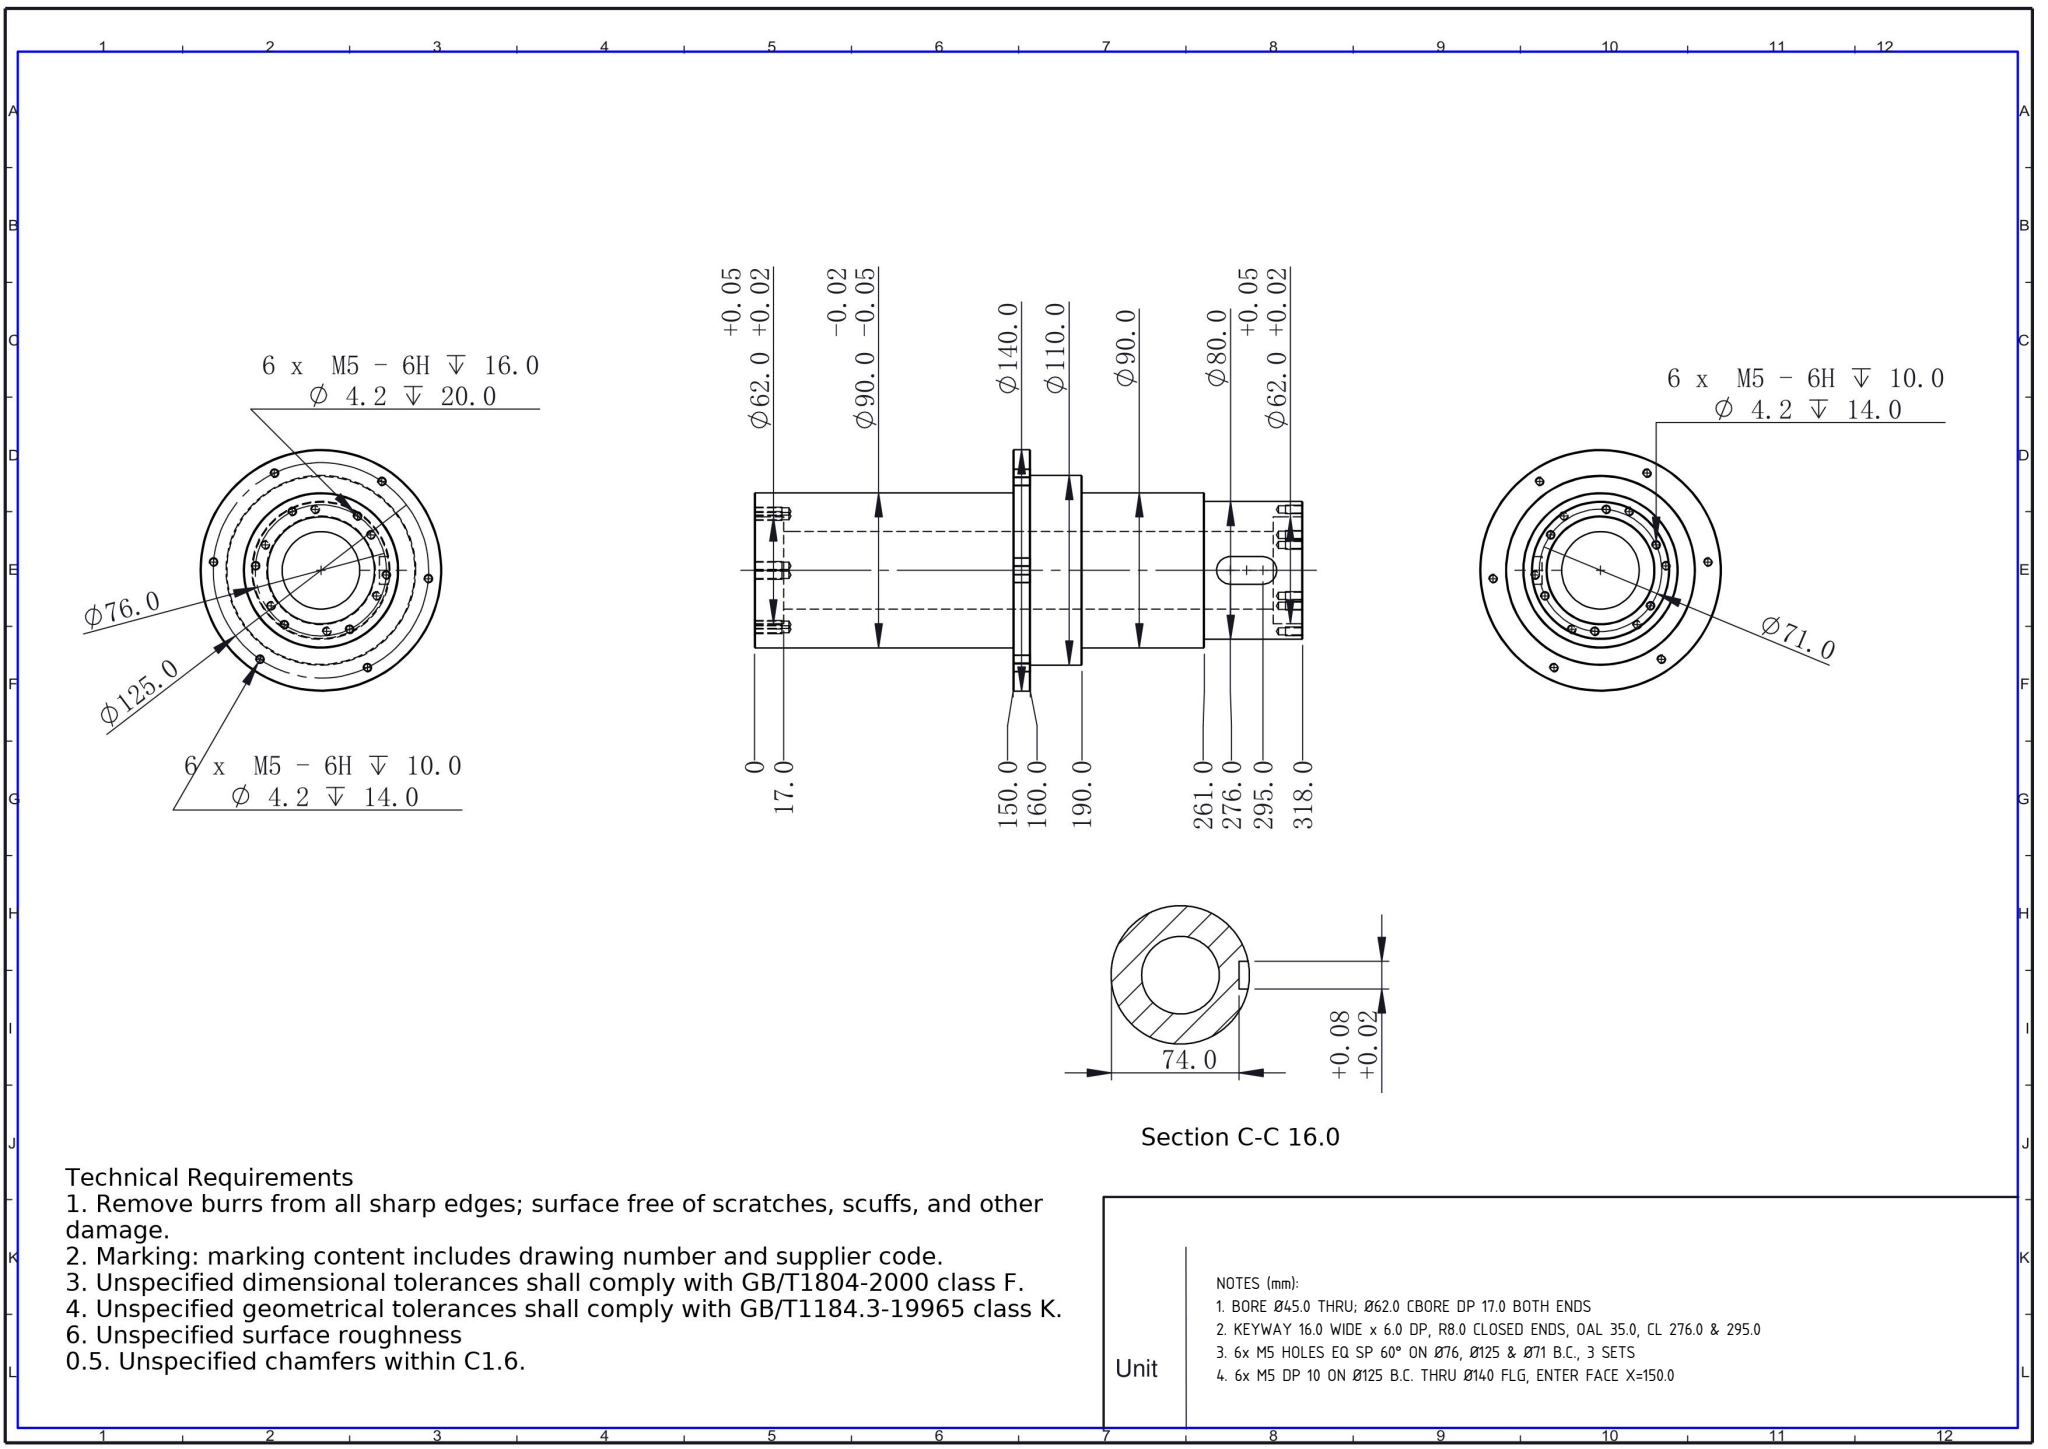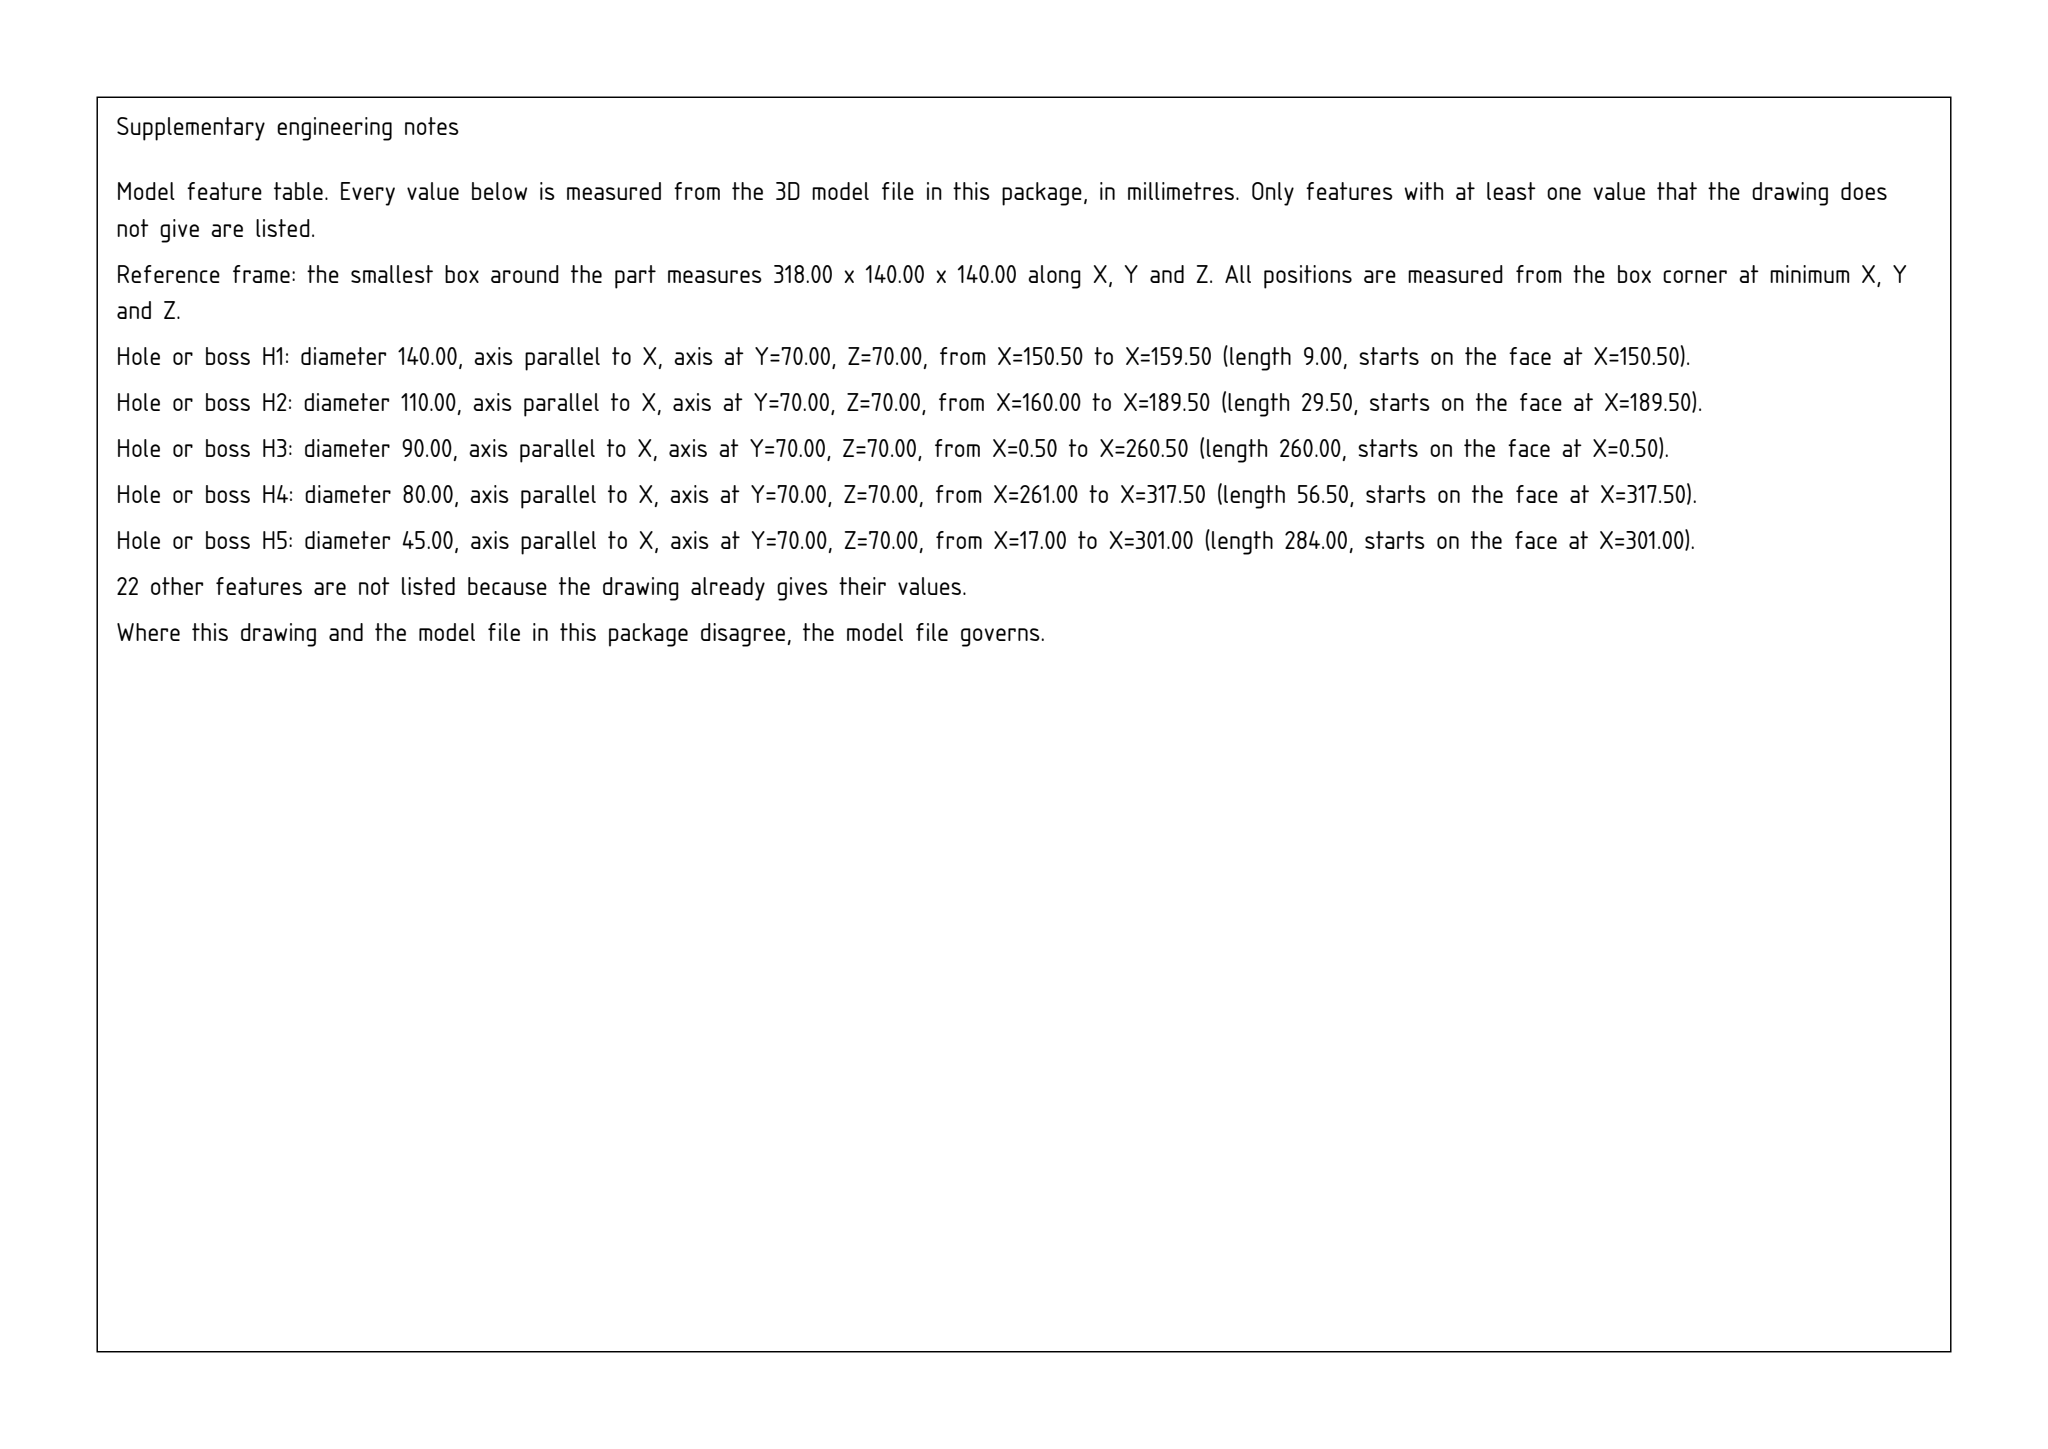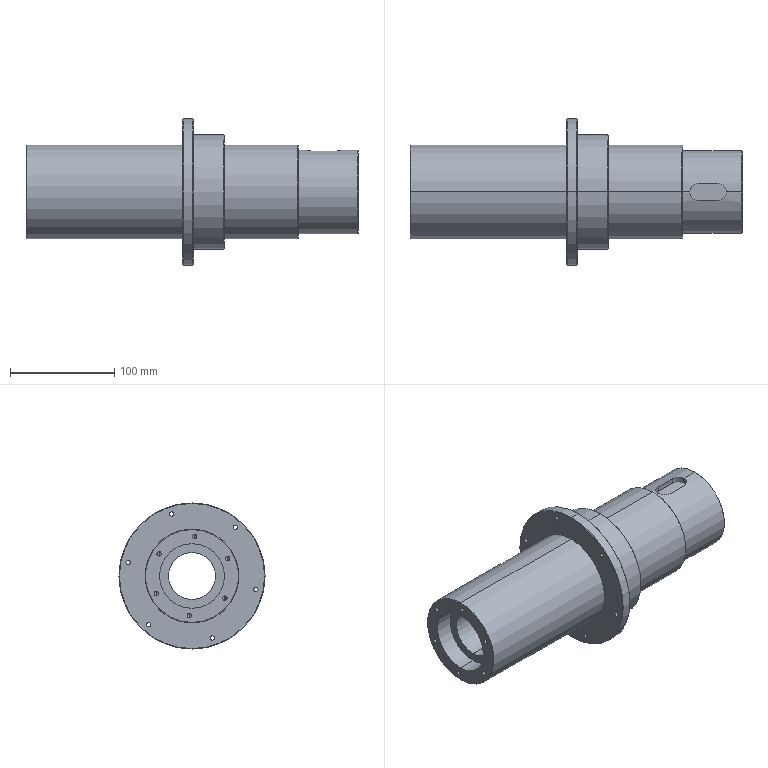Part | SolidWorks | mm | 1 solid | 104 faces | box 318 x 140 x 140 mm | volume 1570246 mm3 | cylinder 55 | cone 38 | plane 11 | commonest cylinder face diameters 4.2 x36 62 x4 90 x4 16 x3 80 x2 110 x2 140 x2 45 x2
Drawing notes:
BORE Ø45.0 THRU; Ø62.0 CBORE DP 17.0 BOTH ENDS | from the solid: Ø45 x-cyl len 284 (x=17 to 301); Ø62 x-cyls at both ends; x-planes 0,17,301,318
KEYWAY 16.0 WIDE x 6.0 DP, R8.0 CLOSED ENDS, OAL 35.0, CL 276.0 & 295.0 | from the solid: y-planes 62.0/78.0 = 16 wide; z-plane 104.0 floor vs Ø80 axis z=70 -> 6 DP; Ø16 z-cyls len 6.0 at x=276.0 & 295.0 -> 19+16=35 OAL
6x M5 HOLES EQ SP 60° ON Ø76, Ø125 & Ø71 B.C., 3 SETS | from the solid: Ø4.2 groups of 6: L=20 at r=38.0, L=10 at r=62.5, L=14 at r=35.5, all 60° increments about axis y=z=70
6x M5 DP 10 ON Ø125 B.C. THRU Ø140 FLG, ENTER FACE X=150.0 | from the solid: Ø4.2 L=10.0 holes at r=62.5 lie in Ø140 flange between x-planes 150.0 and 160.0; hole len = flange thk
build123d program:
from build123d import *

# Parameters (mm, degrees)
CUT_EXTRUDE1_DEPTH    = 6
M5_TAPPED_HOLE1_D     = 4.2
M5_TAPPED_HOLE1_DEPTH = 14
M5_TAPPED_HOLE1_TIP   = 1.262
M5_TAPPED_HOLE2_D     = 4.2
M5_TAPPED_HOLE2_DEPTH = 14
M5_TAPPED_HOLE2_TIP   = 1.262
M5_TAPPED_HOLE3_D     = 4.2
M5_TAPPED_HOLE3_DEPTH = 20
M5_TAPPED_HOLE3_TIP   = 1.262
CHAMFER1_SIZE         = 0.5


with BuildPart() as part:
    # Sketch1 → Revolve1 (revolve)
    with BuildSketch(Plane.XY, mode=Mode.PRIVATE) as revolve1_sk:
        Polygon((17, 22.5), (17, 31), (0, 31), (0, 45), (150, 45), (150, 70), (160, 70), (160, 55), (190, 55), (190, 45), (261, 45), (261, 40), (318, 40), (318, 31), (301, 31), (301, 22.5), align=None)
    revolve(revolve1_sk.sketch.rotate(Axis((0, 0, 0), (1, 0, 0)), 90), axis=Axis((0, 0, 0), (1, 0, 0)))

    # Sketch2 → Cut-Extrude1 (cut)
    with BuildSketch(Plane.XY.offset(40)):
        with BuildLine():
            Line((276, 8), (295, 8))
            ThreePointArc((295, 8), (303, 0), (295, -8))
            Line((295, -8), (276, -8))
            ThreePointArc((276, -8), (268, 0), (276, 8))
        make_face()
    extrude(amount=-CUT_EXTRUDE1_DEPTH, mode=Mode.SUBTRACT)

    # M5 Tapped Hole1
    with Locations(Plane(origin=(318, 0, 0), x_dir=(0, 0, -1), z_dir=(1, 0, 0))):
        with Locations((-32.272, -14.791), (-28.945, 20.553), (3.327, 35.344), (32.272, 14.791), (28.945, -20.553), (-3.327, -35.344)):
            Hole(M5_TAPPED_HOLE1_D / 2, depth=M5_TAPPED_HOLE1_DEPTH)
            with Locations((0, 0, -(M5_TAPPED_HOLE1_DEPTH + M5_TAPPED_HOLE1_TIP / 2))):  # 118° drill point
                Cone(0, M5_TAPPED_HOLE1_D / 2, M5_TAPPED_HOLE1_TIP, mode=Mode.SUBTRACT)

    # M5 Tapped Hole2
    with Locations(Plane.ZY.offset(-150)):
        with Locations((46.627, -41.62), (59.357, 19.57), (12.73, 61.19), (-46.627, 41.62), (-59.357, -19.57), (-12.73, -61.19)):
            Hole(M5_TAPPED_HOLE2_D / 2, depth=M5_TAPPED_HOLE2_DEPTH)
            with Locations((0, 0, -(M5_TAPPED_HOLE2_DEPTH + M5_TAPPED_HOLE2_TIP / 2))):  # 118° drill point
                Cone(0, M5_TAPPED_HOLE2_D / 2, M5_TAPPED_HOLE2_TIP, mode=Mode.SUBTRACT)

    # M5 Tapped Hole3
    with Locations(Plane.ZY):
        with Locations((-16.661, 34.153), (-37.908, 2.647), (21.246, 31.506), (37.908, -2.647), (16.661, -34.153), (-21.246, -31.506)):
            Hole(M5_TAPPED_HOLE3_D / 2, depth=M5_TAPPED_HOLE3_DEPTH)
            with Locations((0, 0, -(M5_TAPPED_HOLE3_DEPTH + M5_TAPPED_HOLE3_TIP / 2))):  # 118° drill point
                Cone(0, M5_TAPPED_HOLE3_D / 2, M5_TAPPED_HOLE3_TIP, mode=Mode.SUBTRACT)

    # Chamfer1
    chamfer1_edges = [part.edges().sort_by_distance(p)[0] for p in [
        (318, 0, -31),
        (318, 0, -40),
        (261, 0, -45),
        (190, 0, -55),
        (160, 0, -70),
        (150, 0, -70),
        (0, 0, -45),
    ]]
    chamfer(chamfer1_edges, length=CHAMFER1_SIZE)


solid = part.part